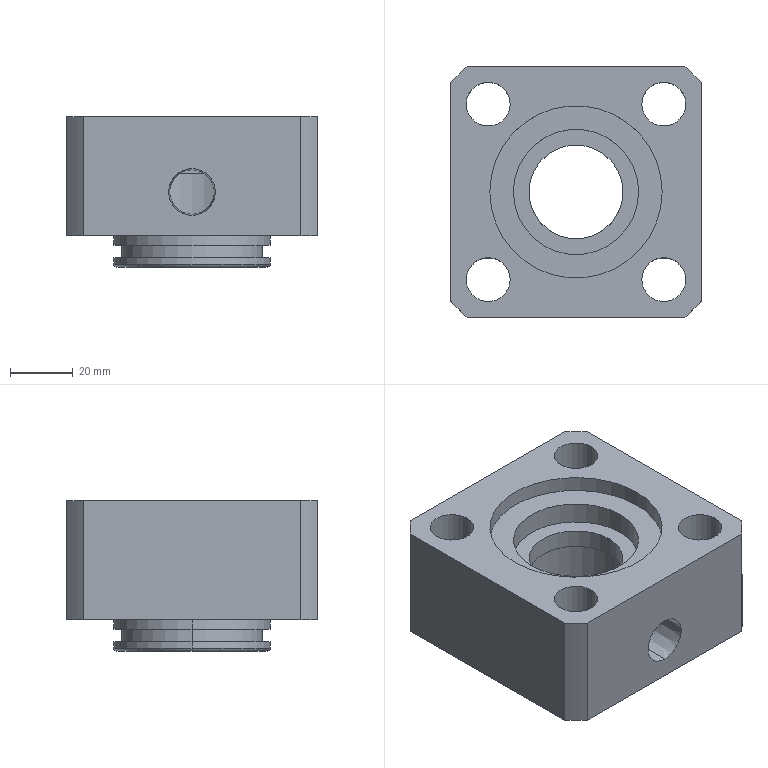Component | SolidWorks | Cylinder-1_FrontEndCap-1 | 1 solid | 45 faces | box 80 x 80 x 48 mm | volume 178384 mm3 | cylinder 28 | plane 13 | torus 2 | cone 2 | commonest cylinder face diameters 14 x8 50 x4 106 x4 14.3 x2 45 x2 35 x2 55 x2 40 x2
build123d program:
from build123d import *

# Parameters (mm, degrees)
SKETCH1_W           = 80
SKETCH1_H           = 80
BOSS_EXTRUDE1_DEPTH = 48
SKETCH2_R           = 15
CUT_EXTRUDE1_DEPTH  = 48
SKETCH4_R           = 20
CUT_EXTRUDE2_DEPTH  = 12
SKETCH5_R           = 27.5
CUT_EXTRUDE3_DEPTH  = 5
SKETCH6_R           = 17.5
CUT_EXTRUDE4_DEPTH  = 30
SKETCH7_R           = 7
CUT_EXTRUDE5_DEPTH  = 48
SKETCH11_OUTSIDE_W  = 106.58
SKETCH11_OUTSIDE_H  = 106.58
SKETCH11_OUTSIDE_R  = 53
CUT_EXTRUDE6_DEPTH  = 123.898
FILLET1_R           = 1


with BuildPart() as part:
    # Sketch1 → Boss-Extrude1 (new body)
    with BuildSketch(Plane.XY):
        with Locations((40, 40)):
            Rectangle(SKETCH1_W, SKETCH1_H)
    extrude(amount=BOSS_EXTRUDE1_DEPTH)

    # Sketch2 → Cut-Extrude1 (cut)
    with BuildSketch(Plane.XY.offset(48)):
        with Locations((40, 40)):
            Circle(SKETCH2_R)
    extrude(amount=-CUT_EXTRUDE1_DEPTH, mode=Mode.SUBTRACT)

    # Sketch4 → Cut-Extrude2 (cut)
    with BuildSketch(Plane.XY.offset(48)):
        with Locations((40, 40)):
            Circle(SKETCH4_R)
    extrude(amount=-CUT_EXTRUDE2_DEPTH, mode=Mode.SUBTRACT)

    # Sketch5 → Cut-Extrude3 (cut)
    with BuildSketch(Plane.XY.offset(48)):
        with Locations((40, 40)):
            Circle(SKETCH5_R)
    extrude(amount=-CUT_EXTRUDE3_DEPTH, mode=Mode.SUBTRACT)

    # Sketch6 → Cut-Extrude4 (cut)
    with BuildSketch(Plane(origin=(0, 0, 0), x_dir=(-1, 0, 0), z_dir=(0, 0, -1))):
        with Locations((-40, 40)):
            Circle(SKETCH6_R)
    extrude(amount=-CUT_EXTRUDE4_DEPTH, mode=Mode.SUBTRACT)

    # Sketch7 → Cut-Extrude5 (cut)
    with BuildSketch(Plane.XY.offset(48)):
        with Locations((12, 68)):
            Circle(SKETCH7_R)
        with Locations(Location((68, 68, 0), (0, 0, 180))):
            Circle(SKETCH7_R)
        with Locations((68, 12)):
            Circle(SKETCH7_R)
        with Locations(Location((12, 12, 0), (0, 0, 180))):
            Circle(SKETCH7_R)
    extrude(amount=-CUT_EXTRUDE5_DEPTH, mode=Mode.SUBTRACT)

    # Sketch8 → Cut-Revolve4 (revolve, cut)
    with BuildSketch(Plane(origin=(40, 0, 0), x_dir=(0, 0, -1), z_dir=(1, 0, 0)), mode=Mode.PRIVATE) as cut_revolve4_sk:
        Polygon((0, 65), (-3, 65), (-3, 62.5), (-7, 62.5), (-7, 65), (-10, 65), (-10, 112.5), (0, 112.5), (0, 80), align=None)
    revolve(cut_revolve4_sk.sketch.rotate(Axis((40, 40, 48), (0, 0, -1)), 90), axis=Axis((40, 40, 48), (0, 0, -1)), mode=Mode.SUBTRACT)

    # Sketch9 → 3_8 Rc Tapped Hole1 (revolve, cut)
    with BuildSketch(Plane(origin=(40, 80, 24), x_dir=(0, 0, 1), z_dir=(1, 0, 0))):
        Polygon((0, 0), (0, 32.386), (7.15, 28.09), (7.15, 11.4), (7.119, 11.4), (7.475, 0), align=None)
    revolve(axis=Axis((40, 86.35, 24), (0, -1, 0)), mode=Mode.SUBTRACT)

    # Sketch11 outside → Cut-Extrude6 (cut, through all)
    with BuildSketch(Plane.XY.offset(48)):
        with Locations((40, 40)):
            Rectangle(SKETCH11_OUTSIDE_W, SKETCH11_OUTSIDE_H)
        with Locations((40, 40)):
            Circle(SKETCH11_OUTSIDE_R, mode=Mode.SUBTRACT)
    extrude(amount=-CUT_EXTRUDE6_DEPTH, mode=Mode.SUBTRACT)

    # Fillet1
    fillet1_edges = [part.edges().sort_by_distance(p)[0] for p in [
        (15, 40, 0),
    ]]
    fillet(fillet1_edges, radius=FILLET1_R)


solid = part.part

# Placed as in the assembly
solid = solid.moved(Location((-140.557, 66.412, -242.351), (0, 0, 180)))